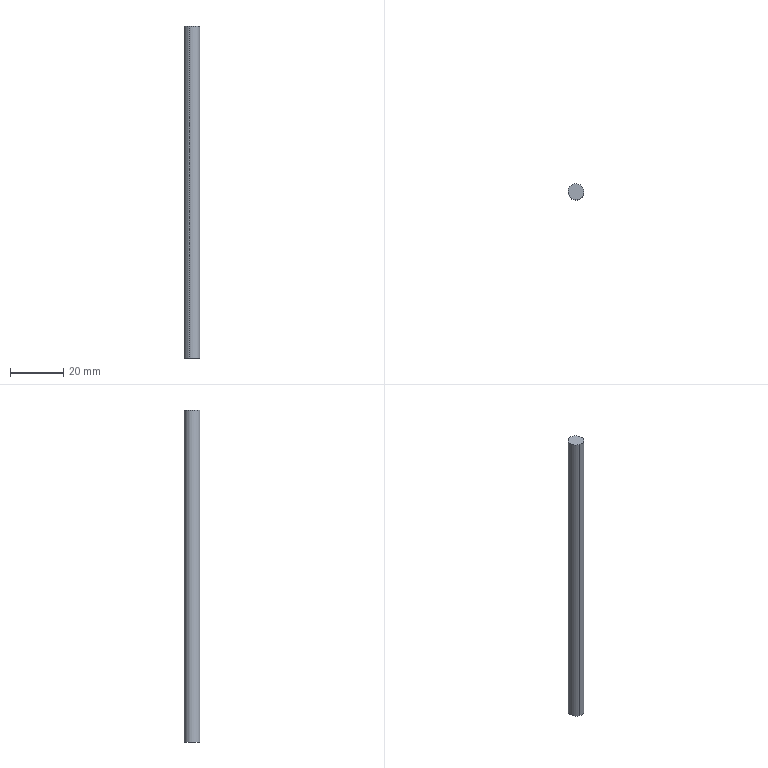Component | SolidWorks | TAR-02-035TieRod-1 | 1 solid | 4 faces | box 6 x 6 x 125 mm | volume 3534 mm3 | cylinder 2 | plane 2 | commonest cylinder face diameters 6 x2
build123d program:
from build123d import *

# Parameters (mm, degrees)
SKETCH1_R           = 3
BOSS_EXTRUDE1_DEPTH = 125


with BuildPart() as part:
    # Sketch1 → Boss-Extrude1 (new body)
    with BuildSketch(Plane.XY):
        Circle(SKETCH1_R)
    extrude(amount=BOSS_EXTRUDE1_DEPTH)


solid = part.part

# Placed as in the assembly
solid = solid.moved(Location((-27.816, 60.226, -149.44), (0, 0, 0)))
STEP:
#1=COLOUR_RGB('',0.7922,0.8196,0.9333);
#2=FILL_AREA_STYLE_COLOUR('',#1);
#3=FILL_AREA_STYLE('',(#2));
#4=SURFACE_STYLE_FILL_AREA(#3);
#5=SURFACE_SIDE_STYLE('',(#4));
#6=SURFACE_STYLE_USAGE(.BOTH.,#5);
#7=PRESENTATION_STYLE_ASSIGNMENT((#6));
#8=CARTESIAN_POINT('',(-1.058,2.483,-0.9622));
#9=VERTEX_POINT('',#8);
#10=CARTESIAN_POINT('',(-1.132,2.259,-0.9622));
#11=VERTEX_POINT('',#10);
#12=CARTESIAN_POINT('',(-1.095,2.371,-0.9622));
#13=DIRECTION('',(0.,0.,1.));
#14=DIRECTION('',(0.3158,0.9488,0.));
#15=AXIS2_PLACEMENT_3D('',#12,#13,#14);
#16=CIRCLE('',#15,0.1181);
#17=EDGE_CURVE('',#9,#11,#16,.T.);
#18=ORIENTED_EDGE('',*,*,#17,.F.);
#19=CARTESIAN_POINT('',(-1.058,2.483,-5.883));
#20=VERTEX_POINT('',#19);
#21=CARTESIAN_POINT('',(-1.058,2.483,-0.9622));
#22=DIRECTION('',(0.,0.,-1.));
#23=VECTOR('',#22,39.37);
#24=LINE('',#21,#23);
#25=EDGE_CURVE('',#9,#20,#24,.T.);
#26=ORIENTED_EDGE('',*,*,#25,.T.);
#27=CARTESIAN_POINT('',(-1.132,2.259,-5.883));
#28=VERTEX_POINT('',#27);
#29=CARTESIAN_POINT('',(-1.095,2.371,-5.883));
#30=DIRECTION('',(0.,0.,1.));
#31=DIRECTION('',(0.3158,0.9488,0.));
#32=AXIS2_PLACEMENT_3D('',#29,#30,#31);
#33=CIRCLE('',#32,0.1181);
#34=EDGE_CURVE('',#20,#28,#33,.T.);
#35=ORIENTED_EDGE('',*,*,#34,.T.);
#36=CARTESIAN_POINT('',(-1.132,2.259,-0.9622));
#37=DIRECTION('',(0.,0.,-1.));
#38=VECTOR('',#37,39.37);
#39=LINE('',#36,#38);
#40=EDGE_CURVE('',#11,#28,#39,.T.);
#41=ORIENTED_EDGE('',*,*,#40,.F.);
#42=EDGE_LOOP('',(#18,#26,#35,#41));
#43=FACE_OUTER_BOUND('',#42,.T.);
#44=CARTESIAN_POINT('',(-1.095,2.371,-0.9622));
#45=DIRECTION('',(0.,0.,-1.));
#46=DIRECTION('',(-0.3158,-0.9488,0.));
#47=AXIS2_PLACEMENT_3D('',#44,#45,#46);
#48=CYLINDRICAL_SURFACE('',#47,0.1181);
#49=ADVANCED_FACE('',(#43),#48,.T.);
#50=ORIENTED_EDGE('',*,*,#25,.F.);
#51=CARTESIAN_POINT('',(-1.095,2.371,-0.9622));
#52=DIRECTION('',(0.,0.,1.));
#53=DIRECTION('',(0.3158,0.9488,0.));
#54=AXIS2_PLACEMENT_3D('',#51,#52,#53);
#55=CIRCLE('',#54,0.1181);
#56=EDGE_CURVE('',#11,#9,#55,.T.);
#57=ORIENTED_EDGE('',*,*,#56,.F.);
#58=ORIENTED_EDGE('',*,*,#40,.T.);
#59=CARTESIAN_POINT('',(-1.095,2.371,-5.883));
#60=DIRECTION('',(0.,0.,1.));
#61=DIRECTION('',(0.3158,0.9488,0.));
#62=AXIS2_PLACEMENT_3D('',#59,#60,#61);
#63=CIRCLE('',#62,0.1181);
#64=EDGE_CURVE('',#28,#20,#63,.T.);
#65=ORIENTED_EDGE('',*,*,#64,.T.);
#66=EDGE_LOOP('',(#50,#57,#58,#65));
#67=FACE_OUTER_BOUND('',#66,.T.);
#68=CARTESIAN_POINT('',(-1.095,2.371,-0.9622));
#69=DIRECTION('',(0.,0.,-1.));
#70=DIRECTION('',(-0.3158,-0.9488,0.));
#71=AXIS2_PLACEMENT_3D('',#68,#69,#70);
#72=CYLINDRICAL_SURFACE('',#71,0.1181);
#73=ADVANCED_FACE('',(#67),#72,.T.);
#74=ORIENTED_EDGE('',*,*,#56,.T.);
#75=ORIENTED_EDGE('',*,*,#17,.T.);
#76=EDGE_LOOP('',(#74,#75));
#77=FACE_OUTER_BOUND('',#76,.T.);
#78=CARTESIAN_POINT('',(-1.095,2.371,-0.9622));
#79=DIRECTION('',(0.,0.,1.));
#80=DIRECTION('',(0.3158,0.9488,0.));
#81=AXIS2_PLACEMENT_3D('',#78,#79,#80);
#82=PLANE('',#81);
#83=ADVANCED_FACE('',(#77),#82,.T.);
#84=ORIENTED_EDGE('',*,*,#64,.F.);
#85=ORIENTED_EDGE('',*,*,#34,.F.);
#86=EDGE_LOOP('',(#84,#85));
#87=FACE_OUTER_BOUND('',#86,.T.);
#88=CARTESIAN_POINT('',(-1.095,2.371,-5.883));
#89=DIRECTION('',(0.,0.,1.));
#90=DIRECTION('',(0.3158,0.9488,0.));
#91=AXIS2_PLACEMENT_3D('',#88,#89,#90);
#92=PLANE('',#91);
#93=ADVANCED_FACE('',(#87),#92,.F.);
#94=CLOSED_SHELL('',(#49,#73,#83,#93));
#95=MANIFOLD_SOLID_BREP('',#94);
#96=STYLED_ITEM('',(#7),#95);
#97=PRESENTATION_LAYER_ASSIGNMENT('','',(#96));
#98=CARTESIAN_POINT('',(0.,0.,0.));
#99=DIRECTION('',(0.,0.,1.));
#100=DIRECTION('',(1.,0.,0.));
#101=AXIS2_PLACEMENT_3D('',#98,#99,#100);
#102=(LENGTH_UNIT()NAMED_UNIT(*)SI_UNIT($,.METRE.));
#103=LENGTH_MEASURE_WITH_UNIT(LENGTH_MEASURE(0.0254),#102);
#104=DIMENSIONAL_EXPONENTS(1.,0.,0.,0.,0.,0.,0.);
#105=(CONVERSION_BASED_UNIT('',#103)LENGTH_UNIT()NAMED_UNIT(#104));
#106=UNCERTAINTY_MEASURE_WITH_UNIT(LENGTH_MEASURE(0.00001),#105,'','');
#107=(NAMED_UNIT(*)PLANE_ANGLE_UNIT()SI_UNIT($,.RADIAN.));
#108=(NAMED_UNIT(*)SI_UNIT($,.STERADIAN.)SOLID_ANGLE_UNIT());
#109=(GEOMETRIC_REPRESENTATION_CONTEXT(3)GLOBAL_UNCERTAINTY_ASSIGNED_CONTEXT((#106))GLOBAL_UNIT_ASSIGNED_CONTEXT((#105,#107,#108))REPRESENTATION_CONTEXT('',''));
#110=ADVANCED_BREP_SHAPE_REPRESENTATION('',(#95,#101),#109);
#111=(LENGTH_UNIT()NAMED_UNIT(*)SI_UNIT($,.METRE.));
#112=LENGTH_MEASURE_WITH_UNIT(LENGTH_MEASURE(0.0254),#111);
#113=DIMENSIONAL_EXPONENTS(1.,0.,0.,0.,0.,0.,0.);
#114=(CONVERSION_BASED_UNIT('',#112)LENGTH_UNIT()NAMED_UNIT(#113));
#115=UNCERTAINTY_MEASURE_WITH_UNIT(LENGTH_MEASURE(0.00001),#114,'','');
#116=(NAMED_UNIT(*)PLANE_ANGLE_UNIT()SI_UNIT($,.RADIAN.));
#117=(NAMED_UNIT(*)SI_UNIT($,.STERADIAN.)SOLID_ANGLE_UNIT());
#118=(GEOMETRIC_REPRESENTATION_CONTEXT(3)GLOBAL_UNCERTAINTY_ASSIGNED_CONTEXT((#115))GLOBAL_UNIT_ASSIGNED_CONTEXT((#114,#116,#117))REPRESENTATION_CONTEXT('',''));
#119=MECHANICAL_DESIGN_GEOMETRIC_PRESENTATION_REPRESENTATION('',(#96),#118);